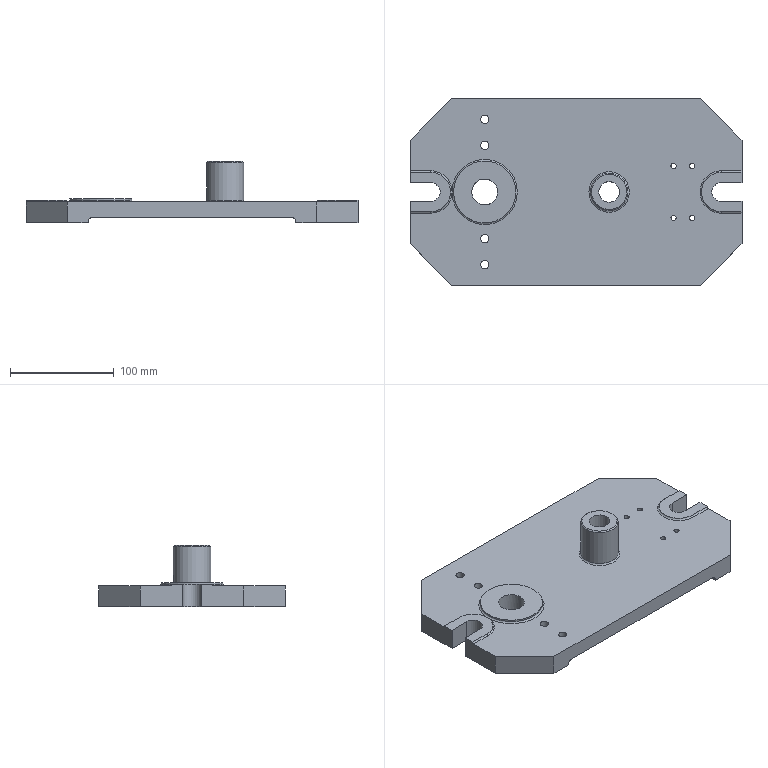Component | NX | FIXTURE_BODY | 1 solid | 59 faces | volume 909993 mm3 | plane 25 | cylinder 25 | torus 4 | cone 3 | spline 2 | commonest cylinder face diameters 8 x9 5 x6 3 x4 18 x2 60 x1 25 x1 36 x1 20 x1